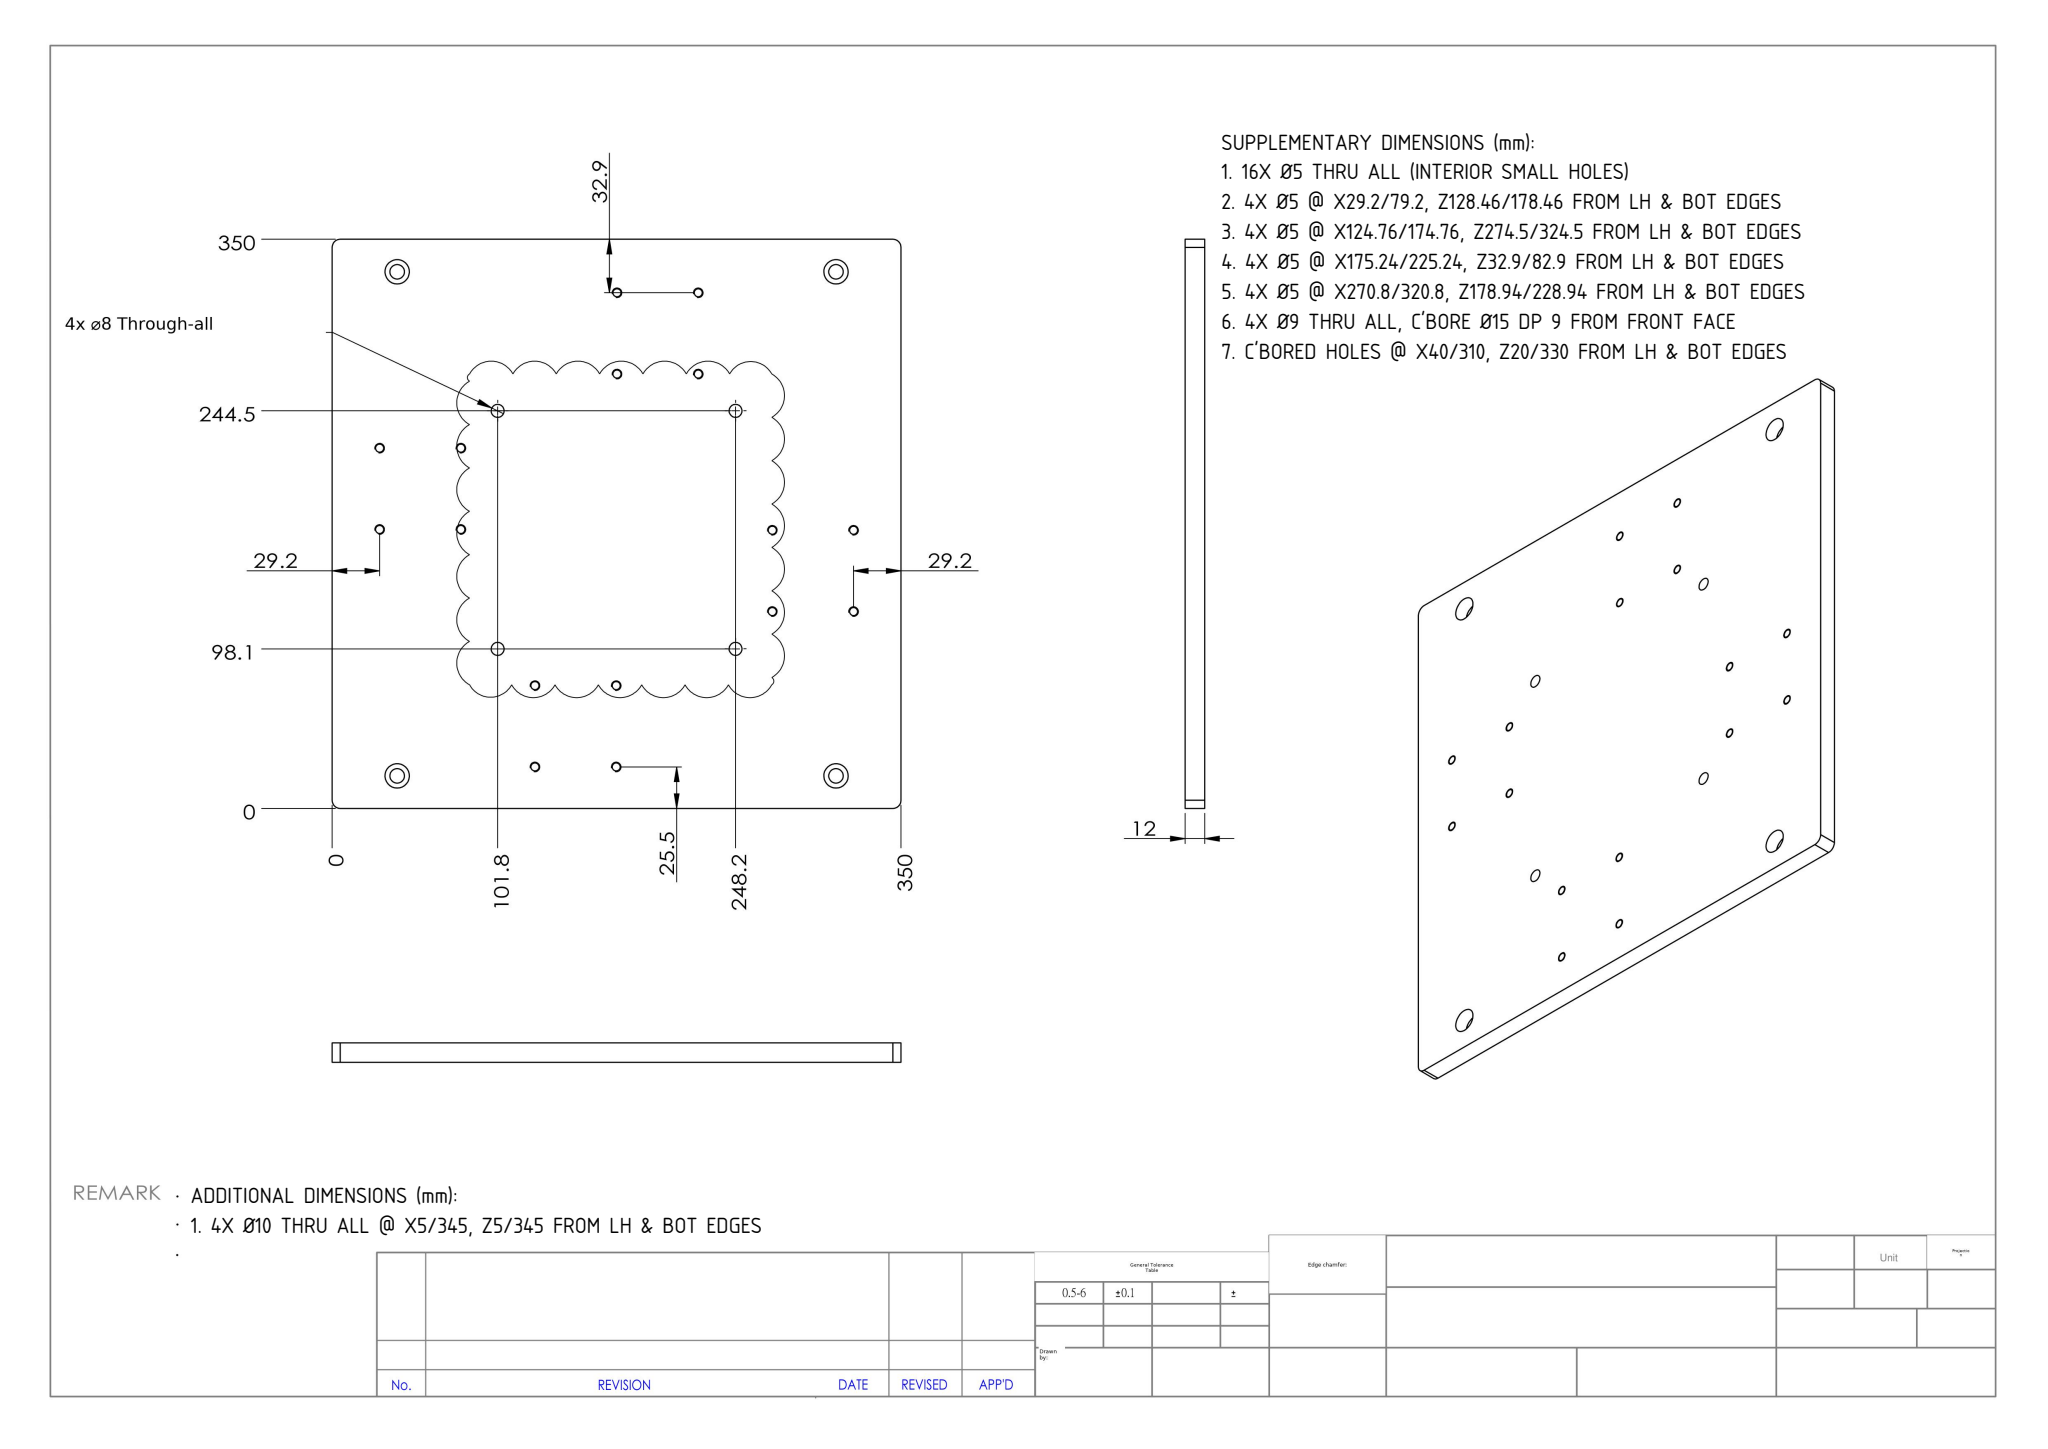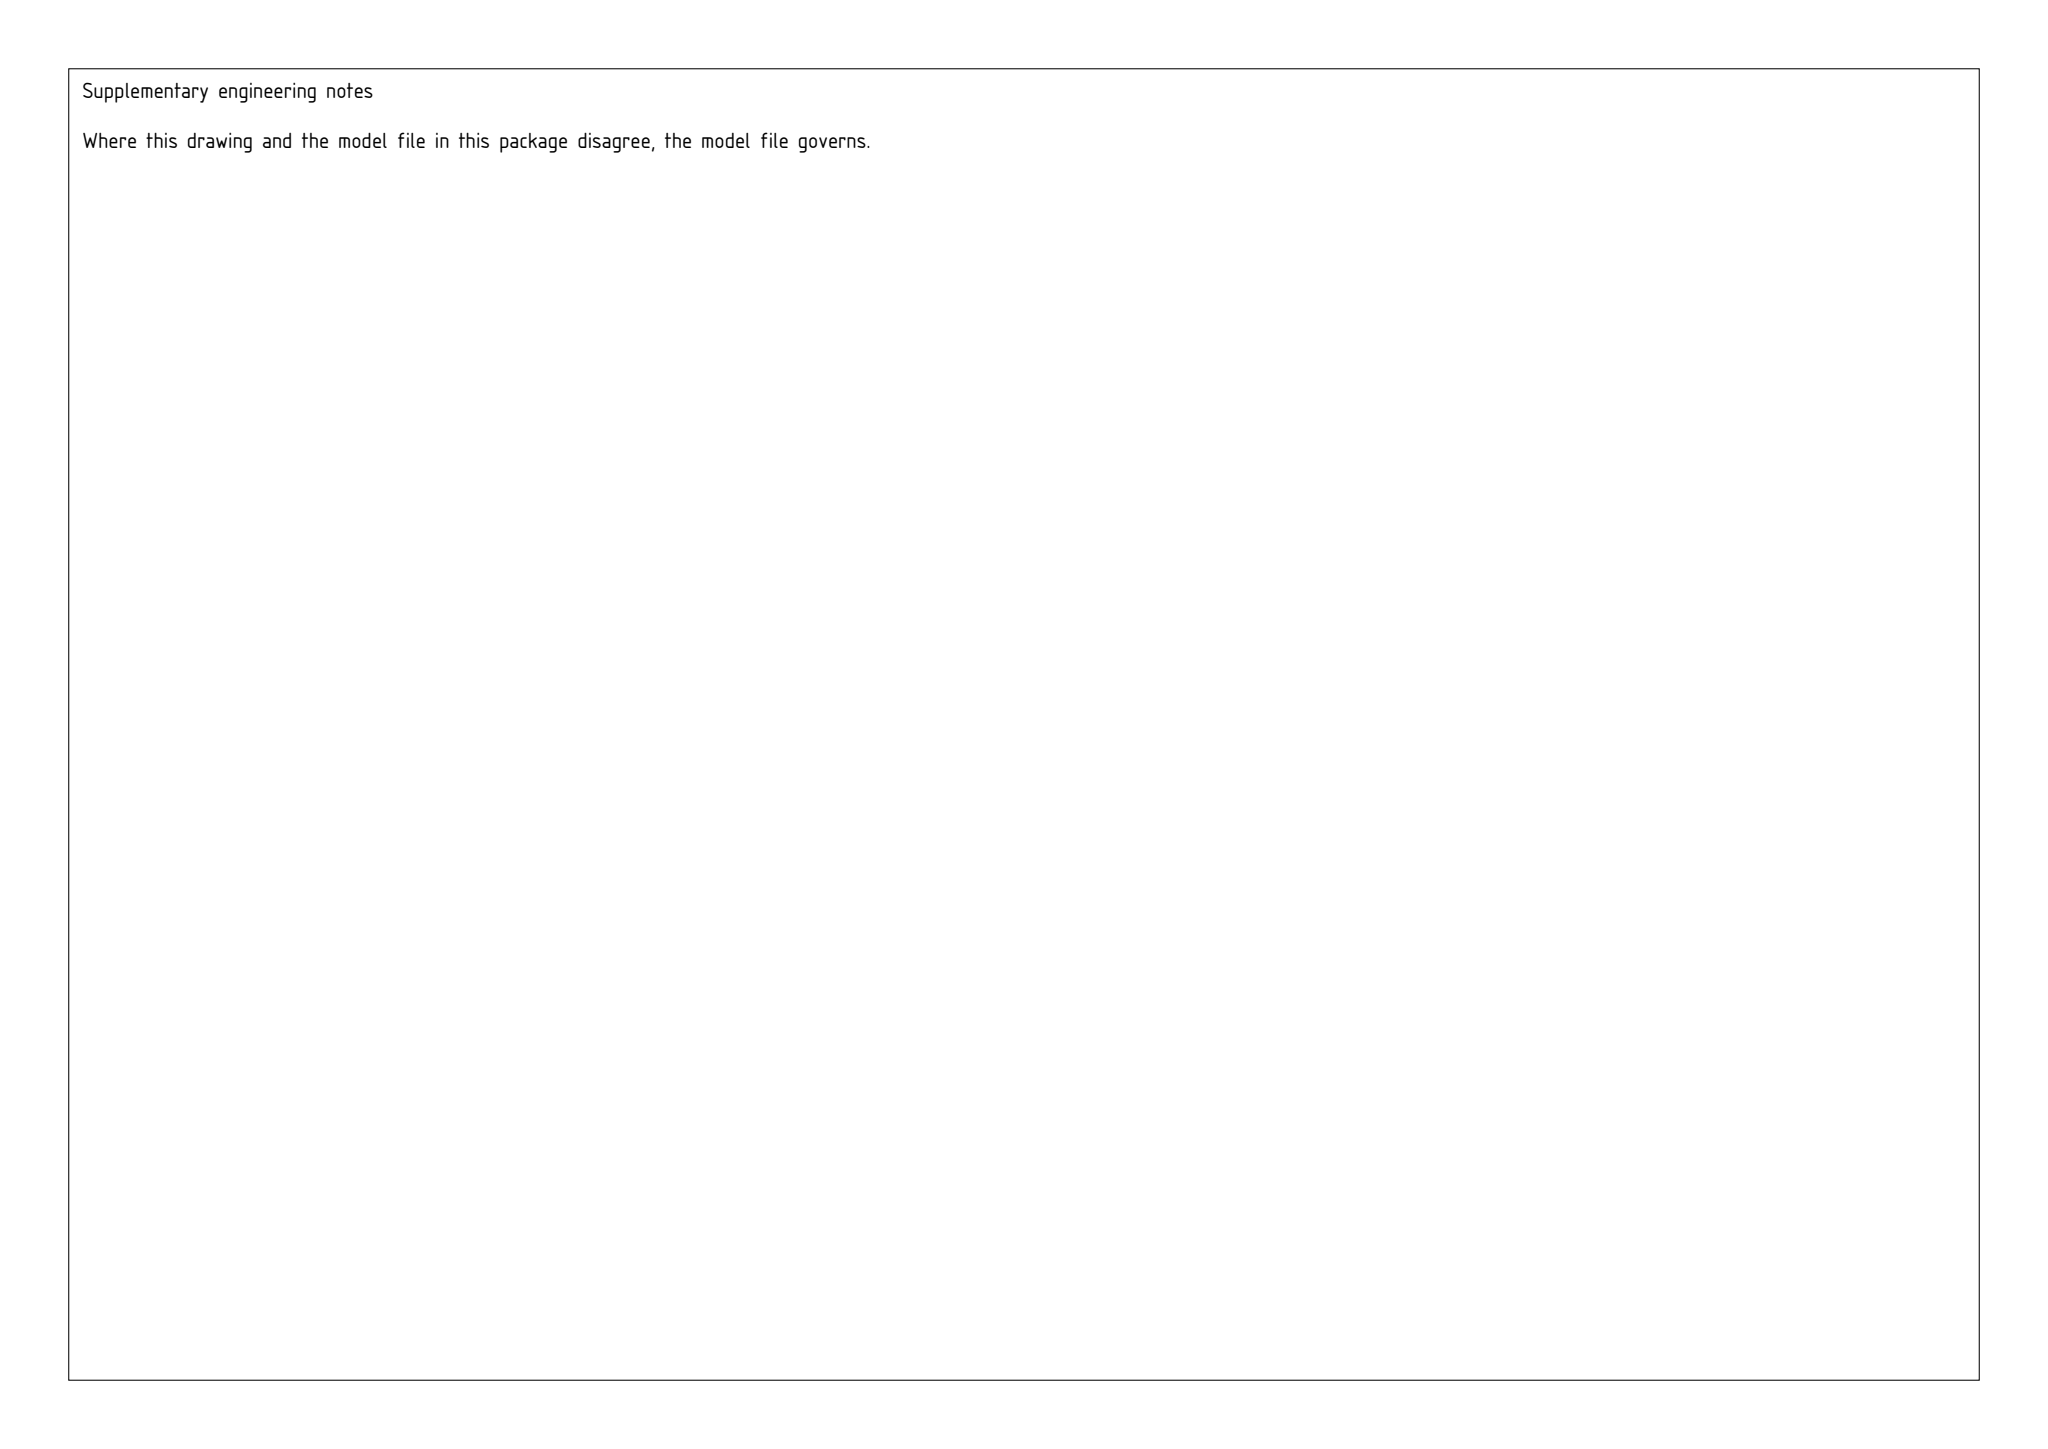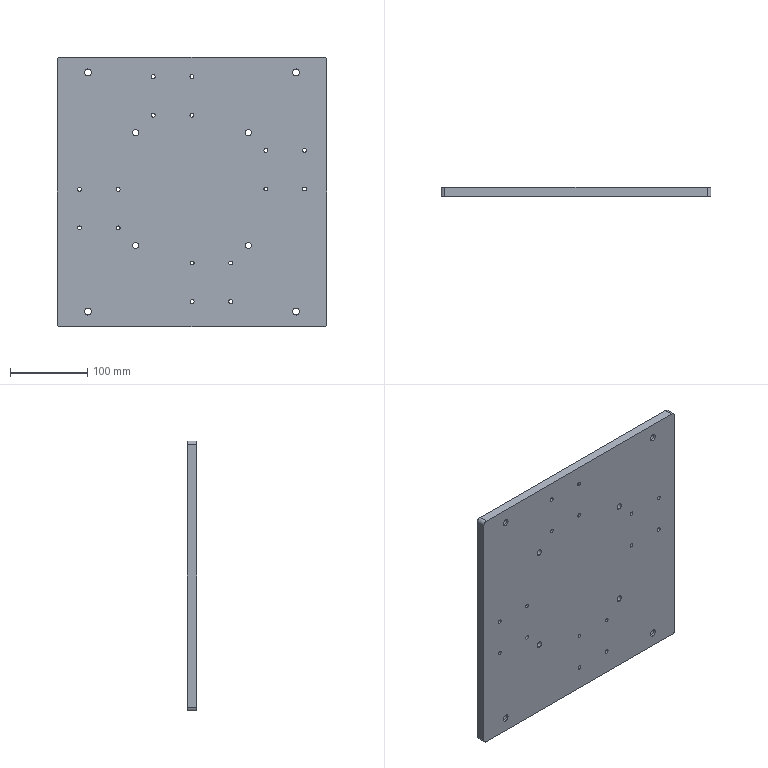Part | SolidWorks | mm | 1 solid | 70 faces | box 350 x 12 x 350 mm | volume 1456435 mm3 | cylinder 60 | plane 10 | commonest cylinder face diameters 5 x32 8 x8 15 x8 9 x8 10 x4
build123d program:
from build123d import *

# Parameters (mm, degrees)
SKETCH1_W                                        = 350
SKETCH1_H                                        = 350
BOSS_EXTRUDE1_DEPTH                              = 12
M6_TAPPED_HOLE1_D                                = 5
FILLET1_R                                        = 5
HOLE_SIZE_BASED_ON_TYPE_1_HEX_SOCKET_D           = 9
HOLE_SIZE_BASED_ON_TYPE_1_HEX_SOCKET_CBORE_D     = 15
HOLE_SIZE_BASED_ON_TYPE_1_HEX_SOCKET_CBORE_DEPTH = 9
M6_CLEARANCE_HOLE_1_D                            = 8


with BuildPart() as part:
    # Sketch1 → Boss-Extrude1 (new body)
    with BuildSketch(Plane(origin=(0, 0, 0), x_dir=(1, 0, 0), z_dir=(0, 1, 0))):
        Rectangle(SKETCH1_W, SKETCH1_H)
    extrude(amount=BOSS_EXTRUDE1_DEPTH)

    # M6 Tapped Hole1 (through all)
    with Locations(Plane(origin=(0, 12, 0), x_dir=(1, 0, 0), z_dir=(0, 1, 0))):
        with Locations((0.2421, 142.1), (95.8, -3.942), (95.8, -53.942), (145.8, -53.942), (145.8, -3.942), (-0.2421, -99.5), (-50.242, -99.5), (-50.242, -149.5), (-0.2421, -149.5), (-95.8, -3.458), (-95.8, 46.542), (-145.8, 46.542), (-145.8, -3.458), (0.2421, 92.1), (50.242, 92.1), (50.242, 142.1)):
            Hole(M6_TAPPED_HOLE1_D / 2)

    # Fillet1
    fillet1_edges = [part.edges().sort_by_distance(p)[0] for p in [
        (175, 6, 175),
        (-175, 6, 175),
        (-175, 6, -175),
        (175, 6, -175),
    ]]
    fillet(fillet1_edges, radius=FILLET1_R)

    # Hole Size _ based on_ Type 1 Hex Socket (through all)
    with Locations(Plane(origin=(0, 12, 0), x_dir=(1, 0, 0), z_dir=(0, 1, 0))):
        with Locations((-135, 155), (135, 155), (135, -155), (-135, -155)):
            CounterBoreHole(HOLE_SIZE_BASED_ON_TYPE_1_HEX_SOCKET_D / 2, HOLE_SIZE_BASED_ON_TYPE_1_HEX_SOCKET_CBORE_D / 2, HOLE_SIZE_BASED_ON_TYPE_1_HEX_SOCKET_CBORE_DEPTH)

    # M6 Clearance Hole 1 (through all)
    with Locations(Plane(origin=(0, 0, 0), x_dir=(-1, 0, 0), z_dir=(0, -1, 0))):
        with Locations((-73.186, 69.487), (-73.186, -76.886), (73.186, -76.886), (73.186, 69.487)):
            Hole(M6_CLEARANCE_HOLE_1_D / 2)


solid = part.part